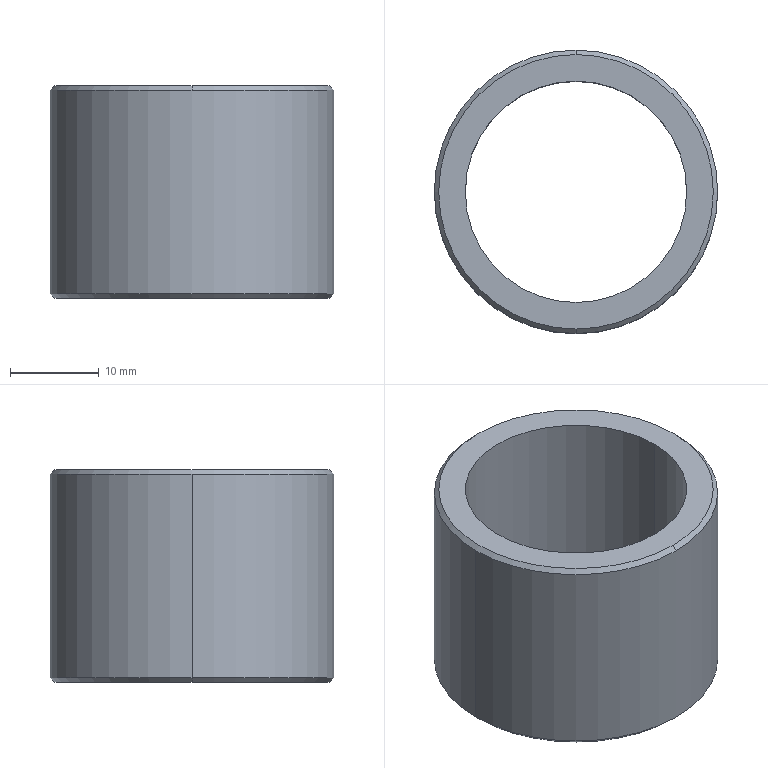Component | SolidWorks | YC1-250-09SecondDropAssembly-1_YC1-25-09-03Collar-1 | 1 solid | 10 faces | box 32 x 32 x 24 mm | volume 7496 mm3 | cylinder 4 | cone 4 | plane 2 | commonest cylinder face diameters 32 x2 25 x2 | material Plain Carbon Steel
STEP:
#1=CARTESIAN_POINT('',(0.,132.323,-38.839));
#2=VERTEX_POINT('',#1);
#3=CARTESIAN_POINT('',(0.6299,131.693,-38.839));
#4=VERTEX_POINT('',#3);
#5=CARTESIAN_POINT('',(0.,131.693,-38.839));
#6=DIRECTION('',(0.,0.,-1.));
#7=DIRECTION('',(-1.,0.,0.));
#8=AXIS2_PLACEMENT_3D('',#5,#6,#7);
#9=CIRCLE('',#8,0.6299);
#10=EDGE_CURVE('',#2,#4,#9,.T.);
#11=ORIENTED_EDGE('',*,*,#10,.T.);
#12=CARTESIAN_POINT('',(0.6299,131.693,-39.744));
#13=VERTEX_POINT('',#12);
#14=CARTESIAN_POINT('',(0.6299,131.693,-38.819));
#15=DIRECTION('',(0.,0.,-1.));
#16=VECTOR('',#15,39.37);
#17=LINE('',#14,#16);
#18=EDGE_CURVE('',#4,#13,#17,.T.);
#19=ORIENTED_EDGE('',*,*,#18,.T.);
#20=CARTESIAN_POINT('',(-0.6299,131.693,-39.744));
#21=VERTEX_POINT('',#20);
#22=CARTESIAN_POINT('',(0.,131.693,-39.744));
#23=DIRECTION('',(0.,0.,1.));
#24=DIRECTION('',(-1.,0.,0.));
#25=AXIS2_PLACEMENT_3D('',#22,#23,#24);
#26=CIRCLE('',#25,0.6299);
#27=EDGE_CURVE('',#13,#21,#26,.T.);
#28=ORIENTED_EDGE('',*,*,#27,.T.);
#29=CARTESIAN_POINT('',(-0.6299,131.693,-38.839));
#30=VERTEX_POINT('',#29);
#31=CARTESIAN_POINT('',(-0.6299,131.693,-38.819));
#32=DIRECTION('',(0.,0.,-1.));
#33=VECTOR('',#32,39.37);
#34=LINE('',#31,#33);
#35=EDGE_CURVE('',#30,#21,#34,.T.);
#36=ORIENTED_EDGE('',*,*,#35,.F.);
#37=CARTESIAN_POINT('',(0.,131.693,-38.839));
#38=DIRECTION('',(0.,0.,-1.));
#39=DIRECTION('',(-1.,0.,0.));
#40=AXIS2_PLACEMENT_3D('',#37,#38,#39);
#41=CIRCLE('',#40,0.6299);
#42=EDGE_CURVE('',#30,#2,#41,.T.);
#43=ORIENTED_EDGE('',*,*,#42,.T.);
#44=EDGE_LOOP('',(#11,#19,#28,#36,#43));
#45=FACE_OUTER_BOUND('',#44,.T.);
#46=CARTESIAN_POINT('',(0.,131.693,-38.819));
#47=DIRECTION('',(0.,0.,-1.));
#48=DIRECTION('',(-1.,0.,0.));
#49=AXIS2_PLACEMENT_3D('',#46,#47,#48);
#50=CYLINDRICAL_SURFACE('',#49,0.6299);
#51=ADVANCED_FACE('',(#45),#50,.T.);
#52=CARTESIAN_POINT('',(0.6102,131.693,-39.764));
#53=VERTEX_POINT('',#52);
#54=CARTESIAN_POINT('',(-0.6102,131.693,-39.764));
#55=VERTEX_POINT('',#54);
#56=CARTESIAN_POINT('',(0.,131.693,-39.764));
#57=DIRECTION('',(0.,0.,1.));
#58=DIRECTION('',(1.,0.,0.));
#59=AXIS2_PLACEMENT_3D('',#56,#57,#58);
#60=CIRCLE('',#59,0.6102);
#61=EDGE_CURVE('',#53,#55,#60,.T.);
#62=ORIENTED_EDGE('',*,*,#61,.T.);
#63=CARTESIAN_POINT('',(-0.6299,131.693,-39.744));
#64=DIRECTION('',(-0.7071,0.,0.7071));
#65=VECTOR('',#64,39.37);
#66=LINE('',#63,#65);
#67=EDGE_CURVE('',#55,#21,#66,.T.);
#68=ORIENTED_EDGE('',*,*,#67,.T.);
#69=ORIENTED_EDGE('',*,*,#27,.F.);
#70=CARTESIAN_POINT('',(0.6299,131.693,-39.744));
#71=DIRECTION('',(0.7071,0.,0.7071));
#72=VECTOR('',#71,39.37);
#73=LINE('',#70,#72);
#74=EDGE_CURVE('',#53,#13,#73,.T.);
#75=ORIENTED_EDGE('',*,*,#74,.F.);
#76=EDGE_LOOP('',(#62,#68,#69,#75));
#77=FACE_OUTER_BOUND('',#76,.T.);
#78=CARTESIAN_POINT('',(0.,131.693,-39.744));
#79=DIRECTION('',(0.,0.,1.));
#80=DIRECTION('',(1.,0.,0.));
#81=AXIS2_PLACEMENT_3D('',#78,#79,#80);
#82=CONICAL_SURFACE('',#81,0.6299,0.7854);
#83=ADVANCED_FACE('',(#77),#82,.T.);
#84=CARTESIAN_POINT('',(0.,132.303,-38.819));
#85=VERTEX_POINT('',#84);
#86=CARTESIAN_POINT('',(0.,131.083,-38.819));
#87=VERTEX_POINT('',#86);
#88=CARTESIAN_POINT('',(0.,131.693,-38.819));
#89=DIRECTION('',(0.,-0.,-1.));
#90=DIRECTION('',(0.,1.,0.));
#91=AXIS2_PLACEMENT_3D('',#88,#89,#90);
#92=CIRCLE('',#91,0.6102);
#93=EDGE_CURVE('',#85,#87,#92,.T.);
#94=ORIENTED_EDGE('',*,*,#93,.T.);
#95=CARTESIAN_POINT('',(0.,131.063,-38.839));
#96=VERTEX_POINT('',#95);
#97=CARTESIAN_POINT('',(0.,131.063,-38.839));
#98=DIRECTION('',(0.,-0.7071,-0.7071));
#99=VECTOR('',#98,39.37);
#100=LINE('',#97,#99);
#101=EDGE_CURVE('',#87,#96,#100,.T.);
#102=ORIENTED_EDGE('',*,*,#101,.T.);
#103=CARTESIAN_POINT('',(0.,131.693,-38.839));
#104=DIRECTION('',(0.,0.,-1.));
#105=DIRECTION('',(-1.,0.,0.));
#106=AXIS2_PLACEMENT_3D('',#103,#104,#105);
#107=CIRCLE('',#106,0.6299);
#108=EDGE_CURVE('',#4,#96,#107,.T.);
#109=ORIENTED_EDGE('',*,*,#108,.F.);
#110=ORIENTED_EDGE('',*,*,#10,.F.);
#111=CARTESIAN_POINT('',(0.,132.323,-38.839));
#112=DIRECTION('',(0.,0.7071,-0.7071));
#113=VECTOR('',#112,39.37);
#114=LINE('',#111,#113);
#115=EDGE_CURVE('',#85,#2,#114,.T.);
#116=ORIENTED_EDGE('',*,*,#115,.F.);
#117=EDGE_LOOP('',(#94,#102,#109,#110,#116));
#118=FACE_OUTER_BOUND('',#117,.T.);
#119=CARTESIAN_POINT('',(0.,131.693,-38.839));
#120=DIRECTION('',(0.,-0.,-1.));
#121=DIRECTION('',(0.,1.,0.));
#122=AXIS2_PLACEMENT_3D('',#119,#120,#121);
#123=CONICAL_SURFACE('',#122,0.6299,0.7854);
#124=ADVANCED_FACE('',(#118),#123,.T.);
#125=CARTESIAN_POINT('',(0.4921,131.693,-38.819));
#126=VERTEX_POINT('',#125);
#127=CARTESIAN_POINT('',(-0.4921,131.693,-38.819));
#128=VERTEX_POINT('',#127);
#129=CARTESIAN_POINT('',(0.,131.693,-38.819));
#130=DIRECTION('',(0.,0.,-1.));
#131=DIRECTION('',(-1.,0.,0.));
#132=AXIS2_PLACEMENT_3D('',#129,#130,#131);
#133=CIRCLE('',#132,0.4921);
#134=EDGE_CURVE('',#126,#128,#133,.T.);
#135=ORIENTED_EDGE('',*,*,#134,.F.);
#136=CARTESIAN_POINT('',(0.4921,131.693,-39.764));
#137=VERTEX_POINT('',#136);
#138=CARTESIAN_POINT('',(0.4921,131.693,-38.819));
#139=DIRECTION('',(0.,0.,-1.));
#140=VECTOR('',#139,39.37);
#141=LINE('',#138,#140);
#142=EDGE_CURVE('',#126,#137,#141,.T.);
#143=ORIENTED_EDGE('',*,*,#142,.T.);
#144=CARTESIAN_POINT('',(-0.4921,131.693,-39.764));
#145=VERTEX_POINT('',#144);
#146=CARTESIAN_POINT('',(0.,131.693,-39.764));
#147=DIRECTION('',(0.,0.,-1.));
#148=DIRECTION('',(-1.,0.,0.));
#149=AXIS2_PLACEMENT_3D('',#146,#147,#148);
#150=CIRCLE('',#149,0.4921);
#151=EDGE_CURVE('',#137,#145,#150,.T.);
#152=ORIENTED_EDGE('',*,*,#151,.T.);
#153=CARTESIAN_POINT('',(-0.4921,131.693,-38.819));
#154=DIRECTION('',(0.,0.,-1.));
#155=VECTOR('',#154,39.37);
#156=LINE('',#153,#155);
#157=EDGE_CURVE('',#128,#145,#156,.T.);
#158=ORIENTED_EDGE('',*,*,#157,.F.);
#159=EDGE_LOOP('',(#135,#143,#152,#158));
#160=FACE_OUTER_BOUND('',#159,.T.);
#161=CARTESIAN_POINT('',(0.,131.693,-38.819));
#162=DIRECTION('',(0.,0.,-1.));
#163=DIRECTION('',(-1.,0.,0.));
#164=AXIS2_PLACEMENT_3D('',#161,#162,#163);
#165=CYLINDRICAL_SURFACE('',#164,0.4921);
#166=ADVANCED_FACE('',(#160),#165,.F.);
#167=ORIENTED_EDGE('',*,*,#18,.F.);
#168=ORIENTED_EDGE('',*,*,#108,.T.);
#169=CARTESIAN_POINT('',(0.,131.693,-38.839));
#170=DIRECTION('',(0.,0.,-1.));
#171=DIRECTION('',(-1.,0.,0.));
#172=AXIS2_PLACEMENT_3D('',#169,#170,#171);
#173=CIRCLE('',#172,0.6299);
#174=EDGE_CURVE('',#96,#30,#173,.T.);
#175=ORIENTED_EDGE('',*,*,#174,.T.);
#176=ORIENTED_EDGE('',*,*,#35,.T.);
#177=CARTESIAN_POINT('',(0.,131.693,-39.744));
#178=DIRECTION('',(0.,0.,1.));
#179=DIRECTION('',(-1.,0.,0.));
#180=AXIS2_PLACEMENT_3D('',#177,#178,#179);
#181=CIRCLE('',#180,0.6299);
#182=EDGE_CURVE('',#21,#13,#181,.T.);
#183=ORIENTED_EDGE('',*,*,#182,.T.);
#184=EDGE_LOOP('',(#167,#168,#175,#176,#183));
#185=FACE_OUTER_BOUND('',#184,.T.);
#186=CARTESIAN_POINT('',(0.,131.693,-38.819));
#187=DIRECTION('',(0.,0.,-1.));
#188=DIRECTION('',(-1.,0.,0.));
#189=AXIS2_PLACEMENT_3D('',#186,#187,#188);
#190=CYLINDRICAL_SURFACE('',#189,0.6299);
#191=ADVANCED_FACE('',(#185),#190,.T.);
#192=ORIENTED_EDGE('',*,*,#67,.F.);
#193=CARTESIAN_POINT('',(0.,131.693,-39.764));
#194=DIRECTION('',(0.,0.,1.));
#195=DIRECTION('',(1.,0.,0.));
#196=AXIS2_PLACEMENT_3D('',#193,#194,#195);
#197=CIRCLE('',#196,0.6102);
#198=EDGE_CURVE('',#55,#53,#197,.T.);
#199=ORIENTED_EDGE('',*,*,#198,.T.);
#200=ORIENTED_EDGE('',*,*,#74,.T.);
#201=ORIENTED_EDGE('',*,*,#182,.F.);
#202=EDGE_LOOP('',(#192,#199,#200,#201));
#203=FACE_OUTER_BOUND('',#202,.T.);
#204=CARTESIAN_POINT('',(0.,131.693,-39.744));
#205=DIRECTION('',(0.,0.,1.));
#206=DIRECTION('',(1.,0.,0.));
#207=AXIS2_PLACEMENT_3D('',#204,#205,#206);
#208=CONICAL_SURFACE('',#207,0.6299,0.7854);
#209=ADVANCED_FACE('',(#203),#208,.T.);
#210=ORIENTED_EDGE('',*,*,#101,.F.);
#211=CARTESIAN_POINT('',(0.,131.693,-38.819));
#212=DIRECTION('',(0.,-0.,-1.));
#213=DIRECTION('',(0.,1.,0.));
#214=AXIS2_PLACEMENT_3D('',#211,#212,#213);
#215=CIRCLE('',#214,0.6102);
#216=EDGE_CURVE('',#87,#85,#215,.T.);
#217=ORIENTED_EDGE('',*,*,#216,.T.);
#218=ORIENTED_EDGE('',*,*,#115,.T.);
#219=ORIENTED_EDGE('',*,*,#42,.F.);
#220=ORIENTED_EDGE('',*,*,#174,.F.);
#221=EDGE_LOOP('',(#210,#217,#218,#219,#220));
#222=FACE_OUTER_BOUND('',#221,.T.);
#223=CARTESIAN_POINT('',(0.,131.693,-38.839));
#224=DIRECTION('',(0.,-0.,-1.));
#225=DIRECTION('',(0.,1.,0.));
#226=AXIS2_PLACEMENT_3D('',#223,#224,#225);
#227=CONICAL_SURFACE('',#226,0.6299,0.7854);
#228=ADVANCED_FACE('',(#222),#227,.T.);
#229=CARTESIAN_POINT('',(0.,131.693,-39.764));
#230=DIRECTION('',(0.,0.,-1.));
#231=DIRECTION('',(-1.,0.,0.));
#232=AXIS2_PLACEMENT_3D('',#229,#230,#231);
#233=CIRCLE('',#232,0.4921);
#234=EDGE_CURVE('',#145,#137,#233,.T.);
#235=ORIENTED_EDGE('',*,*,#234,.F.);
#236=ORIENTED_EDGE('',*,*,#151,.F.);
#237=EDGE_LOOP('',(#235,#236));
#238=FACE_BOUND('',#237,.T.);
#239=ORIENTED_EDGE('',*,*,#61,.F.);
#240=ORIENTED_EDGE('',*,*,#198,.F.);
#241=EDGE_LOOP('',(#239,#240));
#242=FACE_OUTER_BOUND('',#241,.T.);
#243=CARTESIAN_POINT('',(0.,131.693,-39.764));
#244=DIRECTION('',(0.,0.,1.));
#245=DIRECTION('',(1.,0.,0.));
#246=AXIS2_PLACEMENT_3D('',#243,#244,#245);
#247=PLANE('',#246);
#248=ADVANCED_FACE('',(#238,#242),#247,.F.);
#249=CARTESIAN_POINT('',(0.,131.693,-38.819));
#250=DIRECTION('',(0.,0.,-1.));
#251=DIRECTION('',(-1.,0.,0.));
#252=AXIS2_PLACEMENT_3D('',#249,#250,#251);
#253=CIRCLE('',#252,0.4921);
#254=EDGE_CURVE('',#128,#126,#253,.T.);
#255=ORIENTED_EDGE('',*,*,#254,.T.);
#256=ORIENTED_EDGE('',*,*,#134,.T.);
#257=EDGE_LOOP('',(#255,#256));
#258=FACE_BOUND('',#257,.T.);
#259=ORIENTED_EDGE('',*,*,#93,.F.);
#260=ORIENTED_EDGE('',*,*,#216,.F.);
#261=EDGE_LOOP('',(#259,#260));
#262=FACE_OUTER_BOUND('',#261,.T.);
#263=CARTESIAN_POINT('',(0.,131.693,-38.819));
#264=DIRECTION('',(0.,0.,1.));
#265=DIRECTION('',(1.,0.,0.));
#266=AXIS2_PLACEMENT_3D('',#263,#264,#265);
#267=PLANE('',#266);
#268=ADVANCED_FACE('',(#258,#262),#267,.T.);
#269=ORIENTED_EDGE('',*,*,#142,.F.);
#270=ORIENTED_EDGE('',*,*,#254,.F.);
#271=ORIENTED_EDGE('',*,*,#157,.T.);
#272=ORIENTED_EDGE('',*,*,#234,.T.);
#273=EDGE_LOOP('',(#269,#270,#271,#272));
#274=FACE_OUTER_BOUND('',#273,.T.);
#275=CARTESIAN_POINT('',(0.,131.693,-38.819));
#276=DIRECTION('',(0.,0.,-1.));
#277=DIRECTION('',(-1.,0.,0.));
#278=AXIS2_PLACEMENT_3D('',#275,#276,#277);
#279=CYLINDRICAL_SURFACE('',#278,0.4921);
#280=ADVANCED_FACE('',(#274),#279,.F.);
#281=CLOSED_SHELL('',(#51,#83,#124,#166,#191,#209,#228,#248,#268,#280));
#282=MANIFOLD_SOLID_BREP('',#281);
#283=CARTESIAN_POINT('',(0.,0.,0.));
#284=DIRECTION('',(0.,0.,1.));
#285=DIRECTION('',(1.,0.,0.));
#286=AXIS2_PLACEMENT_3D('',#283,#284,#285);
#287=(LENGTH_UNIT()NAMED_UNIT(*)SI_UNIT($,.METRE.));
#288=LENGTH_MEASURE_WITH_UNIT(LENGTH_MEASURE(0.0254),#287);
#289=DIMENSIONAL_EXPONENTS(1.,0.,0.,0.,0.,0.,0.);
#290=(CONVERSION_BASED_UNIT('',#288)LENGTH_UNIT()NAMED_UNIT(#289));
#291=UNCERTAINTY_MEASURE_WITH_UNIT(LENGTH_MEASURE(0.00001),#290,'','');
#292=(NAMED_UNIT(*)PLANE_ANGLE_UNIT()SI_UNIT($,.RADIAN.));
#293=(NAMED_UNIT(*)SI_UNIT($,.STERADIAN.)SOLID_ANGLE_UNIT());
#294=(GEOMETRIC_REPRESENTATION_CONTEXT(3)GLOBAL_UNCERTAINTY_ASSIGNED_CONTEXT((#291))GLOBAL_UNIT_ASSIGNED_CONTEXT((#290,#292,#293))REPRESENTATION_CONTEXT('',''));
#295=ADVANCED_BREP_SHAPE_REPRESENTATION('',(#282,#286),#294);
#296=COLOUR_RGB('',0.7922,0.8196,0.9333);
#297=FILL_AREA_STYLE_COLOUR('',#296);
#298=FILL_AREA_STYLE('',(#297));
#299=SURFACE_STYLE_FILL_AREA(#298);
#300=SURFACE_SIDE_STYLE('',(#299));
#301=SURFACE_STYLE_USAGE(.BOTH.,#300);
#302=PRESENTATION_STYLE_ASSIGNMENT((#301));
#303=STYLED_ITEM('',(#302),#282);
#304=PRESENTATION_LAYER_ASSIGNMENT('','',(#303));
#305=(LENGTH_UNIT()NAMED_UNIT(*)SI_UNIT($,.METRE.));
#306=LENGTH_MEASURE_WITH_UNIT(LENGTH_MEASURE(0.0254),#305);
#307=DIMENSIONAL_EXPONENTS(1.,0.,0.,0.,0.,0.,0.);
#308=(CONVERSION_BASED_UNIT('',#306)LENGTH_UNIT()NAMED_UNIT(#307));
#309=UNCERTAINTY_MEASURE_WITH_UNIT(LENGTH_MEASURE(0.00001),#308,'','');
#310=(NAMED_UNIT(*)PLANE_ANGLE_UNIT()SI_UNIT($,.RADIAN.));
#311=(NAMED_UNIT(*)SI_UNIT($,.STERADIAN.)SOLID_ANGLE_UNIT());
#312=(GEOMETRIC_REPRESENTATION_CONTEXT(3)GLOBAL_UNCERTAINTY_ASSIGNED_CONTEXT((#309))GLOBAL_UNIT_ASSIGNED_CONTEXT((#308,#310,#311))REPRESENTATION_CONTEXT('',''));
#313=MECHANICAL_DESIGN_GEOMETRIC_PRESENTATION_REPRESENTATION('',(#303),#312);